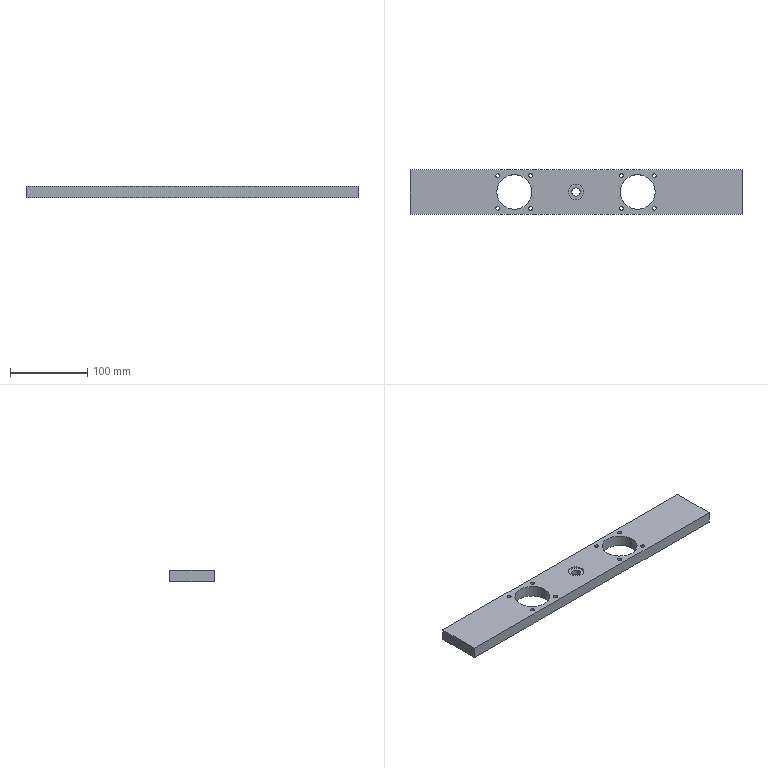Component | SolidWorks | Part19-1 | 1 solid | 31 faces | box 430 x 58 x 15 mm | volume 322167 mm3 | cylinder 24 | plane 7 | commonest cylinder face diameters 5 x16 45 x4 20 x2 11 x2
build123d program:
from build123d import *

# Parameters (mm, degrees)
SKETCH1_W                  = 430
SKETCH1_H                  = 58
BOSS_EXTRUDE1_DEPTH        = 15
SKETCH2_R                  = 5.5
CUT_EXTRUDE1_DEPTH         = 218.465
SKETCH3_R                  = 22.5
CUT_EXTRUDE2_DEPTH         = 218.465
M6_TAPPED_HOLE1_AT_2_COUNT = 2
M6_TAPPED_HOLE1_AT_2_PITCH = 42.426
M6_TAPPED_HOLE1_AT_3_COUNT = 2
M6_TAPPED_HOLE1_AT_3_PITCH = 42.426
M6_TAPPED_HOLE1_AT_4_COUNT = 2
M6_TAPPED_HOLE1_AT_4_PITCH = 60
SKETCH6_R                  = 10
CUT_EXTRUDE3_DEPTH         = 2


with BuildPart() as part:
    # Sketch1 → Boss-Extrude1 (new body)
    with BuildSketch(Plane.XY):
        Rectangle(SKETCH1_W, SKETCH1_H)
    extrude(amount=BOSS_EXTRUDE1_DEPTH)

    # Sketch2 → Cut-Extrude1 (cut, through all)
    with BuildSketch(Plane.XY.offset(15)):
        Circle(SKETCH2_R)
    extrude(amount=-CUT_EXTRUDE1_DEPTH, mode=Mode.SUBTRACT)

    # Sketch3 → Cut-Extrude2 (cut, through all)
    with BuildSketch(Plane.XY.offset(15)):
        with Locations((-80, 0)):
            Circle(SKETCH3_R)
    cut_extrude2 = extrude(amount=-CUT_EXTRUDE2_DEPTH, mode=Mode.SUBTRACT)

    # Sketch5 → M6 Tapped Hole1 (revolve, cut)
    with BuildSketch(Plane(origin=(-101.213, -21.213, 15), x_dir=(0, -1, 0), z_dir=(1, 0, 0))):
        Polygon((0, 0), (0, 16.502), (2.5, 15), (2.5, 0), align=None)
    m6_tapped_hole1 = revolve(axis=Axis((-101.213, -21.213, 21.35), (0, 0, -1)), mode=Mode.SUBTRACT)

    # M6 Tapped Hole1 at 2: M6 Tapped Hole1 ×2
    with Locations(*[(i * M6_TAPPED_HOLE1_AT_2_PITCH, 0, 0) for i in range(1, M6_TAPPED_HOLE1_AT_2_COUNT)]):
        add(m6_tapped_hole1, mode=Mode.SUBTRACT)

    # M6 Tapped Hole1 at 3: M6 Tapped Hole1 ×2
    with Locations(*[(0, i * M6_TAPPED_HOLE1_AT_3_PITCH, 0) for i in range(1, M6_TAPPED_HOLE1_AT_3_COUNT)]):
        add(m6_tapped_hole1, mode=Mode.SUBTRACT)

    # M6 Tapped Hole1 at 4: M6 Tapped Hole1 ×2
    with Locations(*[Vector(0.7071, 0.7071, 0) * (i * M6_TAPPED_HOLE1_AT_4_PITCH) for i in range(1, M6_TAPPED_HOLE1_AT_4_COUNT)]):
        add(m6_tapped_hole1, mode=Mode.SUBTRACT)

    # Mirror1: Cut-Extrude2, M6 Tapped Hole1 across plane
    add(cut_extrude2.mirror(Plane(origin=(0, 0, 0), x_dir=(0, 0, 1), z_dir=(1, 0, 0))), mode=Mode.SUBTRACT)
    add(m6_tapped_hole1.mirror(Plane(origin=(0, 0, 0), x_dir=(0, 0, 1), z_dir=(1, 0, 0))), mode=Mode.SUBTRACT)

    # Mirror1 copy 1 sketch → Mirror1 copy 1 (revolve, cut)
    with BuildSketch(Plane(origin=(58.787, -21.213, 15), x_dir=(0, -1, 0), z_dir=(-1, 0, 0))):
        Polygon((0, 0), (0, -16.502), (2.5, -15), (2.5, 0), align=None)
    revolve(axis=Axis((58.787, -21.213, 21.35), (0, 0, 1)), mode=Mode.SUBTRACT)

    # Mirror1 copy 2 sketch → Mirror1 copy 2 (revolve, cut)
    with BuildSketch(Plane(origin=(101.213, 21.213, 15), x_dir=(0, -1, 0), z_dir=(-1, 0, 0))):
        Polygon((0, 0), (0, -16.502), (2.5, -15), (2.5, 0), align=None)
    revolve(axis=Axis((101.213, 21.213, 21.35), (0, 0, 1)), mode=Mode.SUBTRACT)

    # Mirror1 copy 3 sketch → Mirror1 copy 3 (revolve, cut)
    with BuildSketch(Plane(origin=(58.787, 21.213, 15), x_dir=(0, -1, 0), z_dir=(-1, 0, 0))):
        Polygon((0, 0), (0, -16.502), (2.5, -15), (2.5, 0), align=None)
    revolve(axis=Axis((58.787, 21.213, 21.35), (0, 0, 1)), mode=Mode.SUBTRACT)

    # Sketch6 → Cut-Extrude3 (cut)
    with BuildSketch(Plane.XY.offset(15)):
        Circle(SKETCH6_R)
    extrude(amount=-CUT_EXTRUDE3_DEPTH, mode=Mode.SUBTRACT)


solid = part.part

# Placed as in the assembly
solid = solid.moved(Location((-87.007, -512, -285), (0, 0, 0)))
STEP:
#1=COLOUR_RGB('',0.7922,0.8196,0.9333);
#2=FILL_AREA_STYLE_COLOUR('',#1);
#3=FILL_AREA_STYLE('',(#2));
#4=SURFACE_STYLE_FILL_AREA(#3);
#5=SURFACE_SIDE_STYLE('',(#4));
#6=SURFACE_STYLE_USAGE(.BOTH.,#5);
#7=PRESENTATION_STYLE_ASSIGNMENT((#6));
#8=CARTESIAN_POINT('',(-3.819,-20.157,-10.709));
#9=VERTEX_POINT('',#8);
#10=CARTESIAN_POINT('',(-3.032,-20.157,-10.709));
#11=VERTEX_POINT('',#10);
#12=CARTESIAN_POINT('',(-3.425,-20.157,-10.709));
#13=DIRECTION('',(0.,0.,1.));
#14=DIRECTION('',(1.,0.,0.));
#15=AXIS2_PLACEMENT_3D('',#12,#13,#14);
#16=CIRCLE('',#15,0.3937);
#17=EDGE_CURVE('',#9,#11,#16,.T.);
#18=ORIENTED_EDGE('',*,*,#17,.F.);
#19=CARTESIAN_POINT('',(-3.819,-20.157,-10.63));
#20=VERTEX_POINT('',#19);
#21=CARTESIAN_POINT('',(-3.819,-20.157,-10.709));
#22=DIRECTION('',(0.,0.,1.));
#23=VECTOR('',#22,39.37);
#24=LINE('',#21,#23);
#25=EDGE_CURVE('',#9,#20,#24,.T.);
#26=ORIENTED_EDGE('',*,*,#25,.T.);
#27=CARTESIAN_POINT('',(-3.032,-20.157,-10.63));
#28=VERTEX_POINT('',#27);
#29=CARTESIAN_POINT('',(-3.425,-20.157,-10.63));
#30=DIRECTION('',(0.,0.,1.));
#31=DIRECTION('',(1.,0.,0.));
#32=AXIS2_PLACEMENT_3D('',#29,#30,#31);
#33=CIRCLE('',#32,0.3937);
#34=EDGE_CURVE('',#20,#28,#33,.T.);
#35=ORIENTED_EDGE('',*,*,#34,.T.);
#36=CARTESIAN_POINT('',(-3.032,-20.157,-10.709));
#37=DIRECTION('',(0.,0.,1.));
#38=VECTOR('',#37,39.37);
#39=LINE('',#36,#38);
#40=EDGE_CURVE('',#11,#28,#39,.T.);
#41=ORIENTED_EDGE('',*,*,#40,.F.);
#42=EDGE_LOOP('',(#18,#26,#35,#41));
#43=FACE_OUTER_BOUND('',#42,.T.);
#44=CARTESIAN_POINT('',(-3.425,-20.157,-10.709));
#45=DIRECTION('',(0.,0.,1.));
#46=DIRECTION('',(1.,0.,0.));
#47=AXIS2_PLACEMENT_3D('',#44,#45,#46);
#48=CYLINDRICAL_SURFACE('',#47,0.3937);
#49=ADVANCED_FACE('',(#43),#48,.F.);
#50=CARTESIAN_POINT('',(0.4609,-20.993,-11.22));
#51=VERTEX_POINT('',#50);
#52=CARTESIAN_POINT('',(0.6577,-20.993,-11.22));
#53=VERTEX_POINT('',#52);
#54=CARTESIAN_POINT('',(0.5593,-20.993,-11.22));
#55=DIRECTION('',(0.,0.,1.));
#56=DIRECTION('',(1.,0.,0.));
#57=AXIS2_PLACEMENT_3D('',#54,#55,#56);
#58=CIRCLE('',#57,0.09843);
#59=EDGE_CURVE('',#51,#53,#58,.T.);
#60=ORIENTED_EDGE('',*,*,#59,.F.);
#61=CARTESIAN_POINT('',(0.4609,-20.993,-10.63));
#62=VERTEX_POINT('',#61);
#63=CARTESIAN_POINT('',(0.4609,-20.993,-10.63));
#64=DIRECTION('',(0.,0.,1.));
#65=VECTOR('',#64,39.37);
#66=LINE('',#63,#65);
#67=EDGE_CURVE('',#51,#62,#66,.T.);
#68=ORIENTED_EDGE('',*,*,#67,.T.);
#69=CARTESIAN_POINT('',(0.6577,-20.993,-10.63));
#70=VERTEX_POINT('',#69);
#71=CARTESIAN_POINT('',(0.5593,-20.993,-10.63));
#72=DIRECTION('',(0.,0.,1.));
#73=DIRECTION('',(1.,0.,0.));
#74=AXIS2_PLACEMENT_3D('',#71,#72,#73);
#75=CIRCLE('',#74,0.09843);
#76=EDGE_CURVE('',#62,#70,#75,.T.);
#77=ORIENTED_EDGE('',*,*,#76,.T.);
#78=CARTESIAN_POINT('',(0.6577,-20.993,-10.63));
#79=DIRECTION('',(0.,0.,1.));
#80=VECTOR('',#79,39.37);
#81=LINE('',#78,#80);
#82=EDGE_CURVE('',#53,#70,#81,.T.);
#83=ORIENTED_EDGE('',*,*,#82,.F.);
#84=EDGE_LOOP('',(#60,#68,#77,#83));
#85=FACE_OUTER_BOUND('',#84,.T.);
#86=CARTESIAN_POINT('',(0.5593,-20.993,-10.63));
#87=DIRECTION('',(0.,0.,1.));
#88=DIRECTION('',(1.,0.,0.));
#89=AXIS2_PLACEMENT_3D('',#86,#87,#88);
#90=CYLINDRICAL_SURFACE('',#89,0.09843);
#91=ADVANCED_FACE('',(#85),#90,.F.);
#92=CARTESIAN_POINT('',(-1.209,-20.993,-11.22));
#93=VERTEX_POINT('',#92);
#94=CARTESIAN_POINT('',(-1.013,-20.993,-11.22));
#95=VERTEX_POINT('',#94);
#96=CARTESIAN_POINT('',(-1.111,-20.993,-11.22));
#97=DIRECTION('',(0.,0.,1.));
#98=DIRECTION('',(1.,0.,0.));
#99=AXIS2_PLACEMENT_3D('',#96,#97,#98);
#100=CIRCLE('',#99,0.09843);
#101=EDGE_CURVE('',#93,#95,#100,.T.);
#102=ORIENTED_EDGE('',*,*,#101,.F.);
#103=CARTESIAN_POINT('',(-1.209,-20.993,-10.63));
#104=VERTEX_POINT('',#103);
#105=CARTESIAN_POINT('',(-1.209,-20.993,-10.63));
#106=DIRECTION('',(0.,0.,1.));
#107=VECTOR('',#106,39.37);
#108=LINE('',#105,#107);
#109=EDGE_CURVE('',#93,#104,#108,.T.);
#110=ORIENTED_EDGE('',*,*,#109,.T.);
#111=CARTESIAN_POINT('',(-1.013,-20.993,-10.63));
#112=VERTEX_POINT('',#111);
#113=CARTESIAN_POINT('',(-1.111,-20.993,-10.63));
#114=DIRECTION('',(0.,0.,1.));
#115=DIRECTION('',(1.,0.,0.));
#116=AXIS2_PLACEMENT_3D('',#113,#114,#115);
#117=CIRCLE('',#116,0.09843);
#118=EDGE_CURVE('',#104,#112,#117,.T.);
#119=ORIENTED_EDGE('',*,*,#118,.T.);
#120=CARTESIAN_POINT('',(-1.013,-20.993,-10.63));
#121=DIRECTION('',(0.,0.,1.));
#122=VECTOR('',#121,39.37);
#123=LINE('',#120,#122);
#124=EDGE_CURVE('',#95,#112,#123,.T.);
#125=ORIENTED_EDGE('',*,*,#124,.F.);
#126=EDGE_LOOP('',(#102,#110,#119,#125));
#127=FACE_OUTER_BOUND('',#126,.T.);
#128=CARTESIAN_POINT('',(-1.111,-20.993,-10.63));
#129=DIRECTION('',(0.,0.,1.));
#130=DIRECTION('',(1.,0.,0.));
#131=AXIS2_PLACEMENT_3D('',#128,#129,#130);
#132=CYLINDRICAL_SURFACE('',#131,0.09843);
#133=ADVANCED_FACE('',(#127),#132,.F.);
#134=CARTESIAN_POINT('',(0.4609,-19.322,-11.22));
#135=VERTEX_POINT('',#134);
#136=CARTESIAN_POINT('',(0.6577,-19.322,-11.22));
#137=VERTEX_POINT('',#136);
#138=CARTESIAN_POINT('',(0.5593,-19.322,-11.22));
#139=DIRECTION('',(0.,0.,1.));
#140=DIRECTION('',(1.,0.,0.));
#141=AXIS2_PLACEMENT_3D('',#138,#139,#140);
#142=CIRCLE('',#141,0.09843);
#143=EDGE_CURVE('',#135,#137,#142,.T.);
#144=ORIENTED_EDGE('',*,*,#143,.F.);
#145=CARTESIAN_POINT('',(0.4609,-19.322,-10.63));
#146=VERTEX_POINT('',#145);
#147=CARTESIAN_POINT('',(0.4609,-19.322,-10.63));
#148=DIRECTION('',(0.,0.,1.));
#149=VECTOR('',#148,39.37);
#150=LINE('',#147,#149);
#151=EDGE_CURVE('',#135,#146,#150,.T.);
#152=ORIENTED_EDGE('',*,*,#151,.T.);
#153=CARTESIAN_POINT('',(0.6577,-19.322,-10.63));
#154=VERTEX_POINT('',#153);
#155=CARTESIAN_POINT('',(0.5593,-19.322,-10.63));
#156=DIRECTION('',(0.,0.,1.));
#157=DIRECTION('',(1.,0.,0.));
#158=AXIS2_PLACEMENT_3D('',#155,#156,#157);
#159=CIRCLE('',#158,0.09843);
#160=EDGE_CURVE('',#146,#154,#159,.T.);
#161=ORIENTED_EDGE('',*,*,#160,.T.);
#162=CARTESIAN_POINT('',(0.6577,-19.322,-10.63));
#163=DIRECTION('',(0.,0.,1.));
#164=VECTOR('',#163,39.37);
#165=LINE('',#162,#164);
#166=EDGE_CURVE('',#137,#154,#165,.T.);
#167=ORIENTED_EDGE('',*,*,#166,.F.);
#168=EDGE_LOOP('',(#144,#152,#161,#167));
#169=FACE_OUTER_BOUND('',#168,.T.);
#170=CARTESIAN_POINT('',(0.5593,-19.322,-10.63));
#171=DIRECTION('',(0.,0.,1.));
#172=DIRECTION('',(1.,0.,0.));
#173=AXIS2_PLACEMENT_3D('',#170,#171,#172);
#174=CYLINDRICAL_SURFACE('',#173,0.09843);
#175=ADVANCED_FACE('',(#169),#174,.F.);
#176=CARTESIAN_POINT('',(-1.209,-19.322,-11.22));
#177=VERTEX_POINT('',#176);
#178=CARTESIAN_POINT('',(-1.013,-19.322,-11.22));
#179=VERTEX_POINT('',#178);
#180=CARTESIAN_POINT('',(-1.111,-19.322,-11.22));
#181=DIRECTION('',(0.,0.,1.));
#182=DIRECTION('',(1.,0.,0.));
#183=AXIS2_PLACEMENT_3D('',#180,#181,#182);
#184=CIRCLE('',#183,0.09843);
#185=EDGE_CURVE('',#177,#179,#184,.T.);
#186=ORIENTED_EDGE('',*,*,#185,.F.);
#187=CARTESIAN_POINT('',(-1.209,-19.322,-10.63));
#188=VERTEX_POINT('',#187);
#189=CARTESIAN_POINT('',(-1.209,-19.322,-10.63));
#190=DIRECTION('',(0.,0.,1.));
#191=VECTOR('',#190,39.37);
#192=LINE('',#189,#191);
#193=EDGE_CURVE('',#177,#188,#192,.T.);
#194=ORIENTED_EDGE('',*,*,#193,.T.);
#195=CARTESIAN_POINT('',(-1.013,-19.322,-10.63));
#196=VERTEX_POINT('',#195);
#197=CARTESIAN_POINT('',(-1.111,-19.322,-10.63));
#198=DIRECTION('',(0.,0.,1.));
#199=DIRECTION('',(1.,0.,0.));
#200=AXIS2_PLACEMENT_3D('',#197,#198,#199);
#201=CIRCLE('',#200,0.09843);
#202=EDGE_CURVE('',#188,#196,#201,.T.);
#203=ORIENTED_EDGE('',*,*,#202,.T.);
#204=CARTESIAN_POINT('',(-1.013,-19.322,-10.63));
#205=DIRECTION('',(0.,0.,1.));
#206=VECTOR('',#205,39.37);
#207=LINE('',#204,#206);
#208=EDGE_CURVE('',#179,#196,#207,.T.);
#209=ORIENTED_EDGE('',*,*,#208,.F.);
#210=EDGE_LOOP('',(#186,#194,#203,#209));
#211=FACE_OUTER_BOUND('',#210,.T.);
#212=CARTESIAN_POINT('',(-1.111,-19.322,-10.63));
#213=DIRECTION('',(0.,0.,1.));
#214=DIRECTION('',(1.,0.,0.));
#215=AXIS2_PLACEMENT_3D('',#212,#213,#214);
#216=CYLINDRICAL_SURFACE('',#215,0.09843);
#217=ADVANCED_FACE('',(#211),#216,.F.);
#218=CARTESIAN_POINT('',(0.61,-20.157,-11.22));
#219=VERTEX_POINT('',#218);
#220=CARTESIAN_POINT('',(-1.162,-20.157,-11.22));
#221=VERTEX_POINT('',#220);
#222=CARTESIAN_POINT('',(-0.2759,-20.157,-11.22));
#223=DIRECTION('',(0.,0.,-1.));
#224=DIRECTION('',(-1.,0.,0.));
#225=AXIS2_PLACEMENT_3D('',#222,#223,#224);
#226=CIRCLE('',#225,0.8858);
#227=EDGE_CURVE('',#219,#221,#226,.T.);
#228=ORIENTED_EDGE('',*,*,#227,.T.);
#229=CARTESIAN_POINT('',(-1.162,-20.157,-10.63));
#230=VERTEX_POINT('',#229);
#231=CARTESIAN_POINT('',(-1.162,-20.157,-11.22));
#232=DIRECTION('',(0.,0.,1.));
#233=VECTOR('',#232,39.37);
#234=LINE('',#231,#233);
#235=EDGE_CURVE('',#221,#230,#234,.T.);
#236=ORIENTED_EDGE('',*,*,#235,.T.);
#237=CARTESIAN_POINT('',(0.61,-20.157,-10.63));
#238=VERTEX_POINT('',#237);
#239=CARTESIAN_POINT('',(-0.2759,-20.157,-10.63));
#240=DIRECTION('',(0.,0.,-1.));
#241=DIRECTION('',(-1.,0.,0.));
#242=AXIS2_PLACEMENT_3D('',#239,#240,#241);
#243=CIRCLE('',#242,0.8858);
#244=EDGE_CURVE('',#238,#230,#243,.T.);
#245=ORIENTED_EDGE('',*,*,#244,.F.);
#246=CARTESIAN_POINT('',(0.61,-20.157,-11.22));
#247=DIRECTION('',(0.,0.,1.));
#248=VECTOR('',#247,39.37);
#249=LINE('',#246,#248);
#250=EDGE_CURVE('',#219,#238,#249,.T.);
#251=ORIENTED_EDGE('',*,*,#250,.F.);
#252=EDGE_LOOP('',(#228,#236,#245,#251));
#253=FACE_OUTER_BOUND('',#252,.T.);
#254=CARTESIAN_POINT('',(-0.2759,-20.157,-11.22));
#255=DIRECTION('',(0.,0.,1.));
#256=DIRECTION('',(1.,0.,0.));
#257=AXIS2_PLACEMENT_3D('',#254,#255,#256);
#258=CYLINDRICAL_SURFACE('',#257,0.8858);
#259=ADVANCED_FACE('',(#253),#258,.F.);
#260=CARTESIAN_POINT('',(-7.509,-20.993,-11.22));
#261=VERTEX_POINT('',#260);
#262=CARTESIAN_POINT('',(-7.312,-20.993,-11.22));
#263=VERTEX_POINT('',#262);
#264=CARTESIAN_POINT('',(-7.41,-20.993,-11.22));
#265=DIRECTION('',(0.,0.,1.));
#266=DIRECTION('',(1.,0.,0.));
#267=AXIS2_PLACEMENT_3D('',#264,#265,#266);
#268=CIRCLE('',#267,0.09843);
#269=EDGE_CURVE('',#261,#263,#268,.T.);
#270=ORIENTED_EDGE('',*,*,#269,.F.);
#271=CARTESIAN_POINT('',(-7.509,-20.993,-10.63));
#272=VERTEX_POINT('',#271);
#273=CARTESIAN_POINT('',(-7.509,-20.993,-10.63));
#274=DIRECTION('',(0.,0.,1.));
#275=VECTOR('',#274,39.37);
#276=LINE('',#273,#275);
#277=EDGE_CURVE('',#261,#272,#276,.T.);
#278=ORIENTED_EDGE('',*,*,#277,.T.);
#279=CARTESIAN_POINT('',(-7.312,-20.993,-10.63));
#280=VERTEX_POINT('',#279);
#281=CARTESIAN_POINT('',(-7.41,-20.993,-10.63));
#282=DIRECTION('',(0.,0.,1.));
#283=DIRECTION('',(1.,0.,0.));
#284=AXIS2_PLACEMENT_3D('',#281,#282,#283);
#285=CIRCLE('',#284,0.09843);
#286=EDGE_CURVE('',#272,#280,#285,.T.);
#287=ORIENTED_EDGE('',*,*,#286,.T.);
#288=CARTESIAN_POINT('',(-7.312,-20.993,-10.63));
#289=DIRECTION('',(0.,0.,1.));
#290=VECTOR('',#289,39.37);
#291=LINE('',#288,#290);
#292=EDGE_CURVE('',#263,#280,#291,.T.);
#293=ORIENTED_EDGE('',*,*,#292,.F.);
#294=EDGE_LOOP('',(#270,#278,#287,#293));
#295=FACE_OUTER_BOUND('',#294,.T.);
#296=CARTESIAN_POINT('',(-7.41,-20.993,-10.63));
#297=DIRECTION('',(0.,0.,1.));
#298=DIRECTION('',(1.,0.,0.));
#299=AXIS2_PLACEMENT_3D('',#296,#297,#298);
#300=CYLINDRICAL_SURFACE('',#299,0.09843);
#301=ADVANCED_FACE('',(#295),#300,.F.);
#302=CARTESIAN_POINT('',(-5.838,-20.993,-11.22));
#303=VERTEX_POINT('',#302);
#304=CARTESIAN_POINT('',(-5.641,-20.993,-11.22));
#305=VERTEX_POINT('',#304);
#306=CARTESIAN_POINT('',(-5.74,-20.993,-11.22));
#307=DIRECTION('',(0.,0.,1.));
#308=DIRECTION('',(1.,0.,0.));
#309=AXIS2_PLACEMENT_3D('',#306,#307,#308);
#310=CIRCLE('',#309,0.09843);
#311=EDGE_CURVE('',#303,#305,#310,.T.);
#312=ORIENTED_EDGE('',*,*,#311,.F.);
#313=CARTESIAN_POINT('',(-5.838,-20.993,-10.63));
#314=VERTEX_POINT('',#313);
#315=CARTESIAN_POINT('',(-5.838,-20.993,-10.63));
#316=DIRECTION('',(0.,0.,1.));
#317=VECTOR('',#316,39.37);
#318=LINE('',#315,#317);
#319=EDGE_CURVE('',#303,#314,#318,.T.);
#320=ORIENTED_EDGE('',*,*,#319,.T.);
#321=CARTESIAN_POINT('',(-5.641,-20.993,-10.63));
#322=VERTEX_POINT('',#321);
#323=CARTESIAN_POINT('',(-5.74,-20.993,-10.63));
#324=DIRECTION('',(0.,0.,1.));
#325=DIRECTION('',(1.,0.,0.));
#326=AXIS2_PLACEMENT_3D('',#323,#324,#325);
#327=CIRCLE('',#326,0.09843);
#328=EDGE_CURVE('',#314,#322,#327,.T.);
#329=ORIENTED_EDGE('',*,*,#328,.T.);
#330=CARTESIAN_POINT('',(-5.641,-20.993,-10.63));
#331=DIRECTION('',(0.,0.,1.));
#332=VECTOR('',#331,39.37);
#333=LINE('',#330,#332);
#334=EDGE_CURVE('',#305,#322,#333,.T.);
#335=ORIENTED_EDGE('',*,*,#334,.F.);
#336=EDGE_LOOP('',(#312,#320,#329,#335));
#337=FACE_OUTER_BOUND('',#336,.T.);
#338=CARTESIAN_POINT('',(-5.74,-20.993,-10.63));
#339=DIRECTION('',(0.,0.,1.));
#340=DIRECTION('',(1.,0.,0.));
#341=AXIS2_PLACEMENT_3D('',#338,#339,#340);
#342=CYLINDRICAL_SURFACE('',#341,0.09843);
#343=ADVANCED_FACE('',(#337),#342,.F.);
#344=CARTESIAN_POINT('',(-7.509,-19.322,-11.22));
#345=VERTEX_POINT('',#344);
#346=CARTESIAN_POINT('',(-7.312,-19.322,-11.22));
#347=VERTEX_POINT('',#346);
#348=CARTESIAN_POINT('',(-7.41,-19.322,-11.22));
#349=DIRECTION('',(0.,0.,1.));
#350=DIRECTION('',(1.,0.,0.));
#351=AXIS2_PLACEMENT_3D('',#348,#349,#350);
#352=CIRCLE('',#351,0.09843);
#353=EDGE_CURVE('',#345,#347,#352,.T.);
#354=ORIENTED_EDGE('',*,*,#353,.F.);
#355=CARTESIAN_POINT('',(-7.509,-19.322,-10.63));
#356=VERTEX_POINT('',#355);
#357=CARTESIAN_POINT('',(-7.509,-19.322,-10.63));
#358=DIRECTION('',(0.,0.,1.));
#359=VECTOR('',#358,39.37);
#360=LINE('',#357,#359);
#361=EDGE_CURVE('',#345,#356,#360,.T.);
#362=ORIENTED_EDGE('',*,*,#361,.T.);
#363=CARTESIAN_POINT('',(-7.312,-19.322,-10.63));
#364=VERTEX_POINT('',#363);
#365=CARTESIAN_POINT('',(-7.41,-19.322,-10.63));
#366=DIRECTION('',(0.,0.,1.));
#367=DIRECTION('',(1.,0.,0.));
#368=AXIS2_PLACEMENT_3D('',#365,#366,#367);
#369=CIRCLE('',#368,0.09843);
#370=EDGE_CURVE('',#356,#364,#369,.T.);
#371=ORIENTED_EDGE('',*,*,#370,.T.);
#372=CARTESIAN_POINT('',(-7.312,-19.322,-10.63));
#373=DIRECTION('',(0.,0.,1.));
#374=VECTOR('',#373,39.37);
#375=LINE('',#372,#374);
#376=EDGE_CURVE('',#347,#364,#375,.T.);
#377=ORIENTED_EDGE('',*,*,#376,.F.);
#378=EDGE_LOOP('',(#354,#362,#371,#377));
#379=FACE_OUTER_BOUND('',#378,.T.);
#380=CARTESIAN_POINT('',(-7.41,-19.322,-10.63));
#381=DIRECTION('',(0.,0.,1.));
#382=DIRECTION('',(1.,0.,0.));
#383=AXIS2_PLACEMENT_3D('',#380,#381,#382);
#384=CYLINDRICAL_SURFACE('',#383,0.09843);
#385=ADVANCED_FACE('',(#379),#384,.F.);
#386=CARTESIAN_POINT('',(-5.838,-19.322,-11.22));
#387=VERTEX_POINT('',#386);
#388=CARTESIAN_POINT('',(-5.641,-19.322,-11.22));
#389=VERTEX_POINT('',#388);
#390=CARTESIAN_POINT('',(-5.74,-19.322,-11.22));
#391=DIRECTION('',(0.,0.,1.));
#392=DIRECTION('',(1.,0.,0.));
#393=AXIS2_PLACEMENT_3D('',#390,#391,#392);
#394=CIRCLE('',#393,0.09843);
#395=EDGE_CURVE('',#387,#389,#394,.T.);
#396=ORIENTED_EDGE('',*,*,#395,.F.);
#397=CARTESIAN_POINT('',(-5.838,-19.322,-10.63));
#398=VERTEX_POINT('',#397);
#399=CARTESIAN_POINT('',(-5.838,-19.322,-10.63));
#400=DIRECTION('',(0.,0.,1.));
#401=VECTOR('',#400,39.37);
#402=LINE('',#399,#401);
#403=EDGE_CURVE('',#387,#398,#402,.T.);
#404=ORIENTED_EDGE('',*,*,#403,.T.);
#405=CARTESIAN_POINT('',(-5.641,-19.322,-10.63));
#406=VERTEX_POINT('',#405);
#407=CARTESIAN_POINT('',(-5.74,-19.322,-10.63));
#408=DIRECTION('',(0.,0.,1.));
#409=DIRECTION('',(1.,0.,0.));
#410=AXIS2_PLACEMENT_3D('',#407,#408,#409);
#411=CIRCLE('',#410,0.09843);
#412=EDGE_CURVE('',#398,#406,#411,.T.);
#413=ORIENTED_EDGE('',*,*,#412,.T.);
#414=CARTESIAN_POINT('',(-5.641,-19.322,-10.63));
#415=DIRECTION('',(0.,0.,1.));
#416=VECTOR('',#415,39.37);
#417=LINE('',#414,#416);
#418=EDGE_CURVE('',#389,#406,#417,.T.);
#419=ORIENTED_EDGE('',*,*,#418,.F.);
#420=EDGE_LOOP('',(#396,#404,#413,#419));
#421=FACE_OUTER_BOUND('',#420,.T.);
#422=CARTESIAN_POINT('',(-5.74,-19.322,-10.63));
#423=DIRECTION('',(0.,0.,1.));
#424=DIRECTION('',(1.,0.,0.));
#425=AXIS2_PLACEMENT_3D('',#422,#423,#424);
#426=CYLINDRICAL_SURFACE('',#425,0.09843);
#427=ADVANCED_FACE('',(#421),#426,.F.);
#428=CARTESIAN_POINT('',(-7.461,-20.157,-11.22));
#429=VERTEX_POINT('',#428);
#430=CARTESIAN_POINT('',(-5.689,-20.157,-11.22));
#431=VERTEX_POINT('',#430);
#432=CARTESIAN_POINT('',(-6.575,-20.157,-11.22));
#433=DIRECTION('',(0.,0.,1.));
#434=DIRECTION('',(1.,0.,0.));
#435=AXIS2_PLACEMENT_3D('',#432,#433,#434);
#436=CIRCLE('',#435,0.8858);
#437=EDGE_CURVE('',#429,#431,#436,.T.);
#438=ORIENTED_EDGE('',*,*,#437,.F.);
#439=CARTESIAN_POINT('',(-7.461,-20.157,-10.63));
#440=VERTEX_POINT('',#439);
#441=CARTESIAN_POINT('',(-7.461,-20.157,-11.22));
#442=DIRECTION('',(0.,0.,1.));
#443=VECTOR('',#442,39.37);
#444=LINE('',#441,#443);
#445=EDGE_CURVE('',#429,#440,#444,.T.);
#446=ORIENTED_EDGE('',*,*,#445,.T.);
#447=CARTESIAN_POINT('',(-5.689,-20.157,-10.63));
#448=VERTEX_POINT('',#447);
#449=CARTESIAN_POINT('',(-6.575,-20.157,-10.63));
#450=DIRECTION('',(0.,0.,1.));
#451=DIRECTION('',(1.,0.,0.));
#452=AXIS2_PLACEMENT_3D('',#449,#450,#451);
#453=CIRCLE('',#452,0.8858);
#454=EDGE_CURVE('',#440,#448,#453,.T.);
#455=ORIENTED_EDGE('',*,*,#454,.T.);
#456=CARTESIAN_POINT('',(-5.689,-20.157,-11.22));
#457=DIRECTION('',(0.,0.,1.));
#458=VECTOR('',#457,39.37);
#459=LINE('',#456,#458);
#460=EDGE_CURVE('',#431,#448,#459,.T.);
#461=ORIENTED_EDGE('',*,*,#460,.F.);
#462=EDGE_LOOP('',(#438,#446,#455,#461));
#463=FACE_OUTER_BOUND('',#462,.T.);
#464=CARTESIAN_POINT('',(-6.575,-20.157,-11.22));
#465=DIRECTION('',(0.,0.,1.));
#466=DIRECTION('',(1.,0.,0.));
#467=AXIS2_PLACEMENT_3D('',#464,#465,#466);
#468=CYLINDRICAL_SURFACE('',#467,0.8858);
#469=ADVANCED_FACE('',(#463),#468,.F.);
#470=CARTESIAN_POINT('',(-3.642,-20.157,-11.22));
#471=VERTEX_POINT('',#470);
#472=CARTESIAN_POINT('',(-3.209,-20.157,-11.22));
#473=VERTEX_POINT('',#472);
#474=CARTESIAN_POINT('',(-3.425,-20.157,-11.22));
#475=DIRECTION('',(0.,0.,1.));
#476=DIRECTION('',(1.,0.,0.));
#477=AXIS2_PLACEMENT_3D('',#474,#475,#476);
#478=CIRCLE('',#477,0.2165);
#479=EDGE_CURVE('',#471,#473,#478,.T.);
#480=ORIENTED_EDGE('',*,*,#479,.F.);
#481=CARTESIAN_POINT('',(-3.642,-20.157,-10.709));
#482=VERTEX_POINT('',#481);
#483=CARTESIAN_POINT('',(-3.642,-20.157,-11.22));
#484=DIRECTION('',(0.,0.,1.));
#485=VECTOR('',#484,39.37);
#486=LINE('',#483,#485);
#487=EDGE_CURVE('',#471,#482,#486,.T.);
#488=ORIENTED_EDGE('',*,*,#487,.T.);
#489=CARTESIAN_POINT('',(-3.209,-20.157,-10.709));
#490=VERTEX_POINT('',#489);
#491=CARTESIAN_POINT('',(-3.425,-20.157,-10.709));
#492=DIRECTION('',(0.,0.,-1.));
#493=DIRECTION('',(1.,0.,0.));
#494=AXIS2_PLACEMENT_3D('',#491,#492,#493);
#495=CIRCLE('',#494,0.2165);
#496=EDGE_CURVE('',#490,#482,#495,.T.);
#497=ORIENTED_EDGE('',*,*,#496,.F.);
#498=CARTESIAN_POINT('',(-3.209,-20.157,-11.22));
#499=DIRECTION('',(0.,0.,1.));
#500=VECTOR('',#499,39.37);
#501=LINE('',#498,#500);
#502=EDGE_CURVE('',#473,#490,#501,.T.);
#503=ORIENTED_EDGE('',*,*,#502,.F.);
#504=EDGE_LOOP('',(#480,#488,#497,#503));
#505=FACE_OUTER_BOUND('',#504,.T.);
#506=CARTESIAN_POINT('',(-3.425,-20.157,-11.22));
#507=DIRECTION('',(0.,0.,1.));
#508=DIRECTION('',(1.,0.,0.));
#509=AXIS2_PLACEMENT_3D('',#506,#507,#508);
#510=CYLINDRICAL_SURFACE('',#509,0.2165);
#511=ADVANCED_FACE('',(#505),#510,.F.);
#512=ORIENTED_EDGE('',*,*,#487,.F.);
#513=CARTESIAN_POINT('',(-3.425,-20.157,-11.22));
#514=DIRECTION('',(0.,0.,1.));
#515=DIRECTION('',(1.,0.,0.));
#516=AXIS2_PLACEMENT_3D('',#513,#514,#515);
#517=CIRCLE('',#516,0.2165);
#518=EDGE_CURVE('',#473,#471,#517,.T.);
#519=ORIENTED_EDGE('',*,*,#518,.F.);
#520=ORIENTED_EDGE('',*,*,#502,.T.);
#521=CARTESIAN_POINT('',(-3.425,-20.157,-10.709));
#522=DIRECTION('',(0.,0.,-1.));
#523=DIRECTION('',(1.,0.,0.));
#524=AXIS2_PLACEMENT_3D('',#521,#522,#523);
#525=CIRCLE('',#524,0.2165);
#526=EDGE_CURVE('',#482,#490,#525,.T.);
#527=ORIENTED_EDGE('',*,*,#526,.F.);
#528=EDGE_LOOP('',(#512,#519,#520,#527));
#529=FACE_OUTER_BOUND('',#528,.T.);
#530=CARTESIAN_POINT('',(-3.425,-20.157,-11.22));
#531=DIRECTION('',(0.,0.,1.));
#532=DIRECTION('',(1.,0.,0.));
#533=AXIS2_PLACEMENT_3D('',#530,#531,#532);
#534=CYLINDRICAL_SURFACE('',#533,0.2165);
#535=ADVANCED_FACE('',(#529),#534,.F.);
#536=CARTESIAN_POINT('',(5.039,-21.299,-11.22));
#537=VERTEX_POINT('',#536);
#538=CARTESIAN_POINT('',(5.039,-19.016,-11.22));
#539=VERTEX_POINT('',#538);
#540=CARTESIAN_POINT('',(5.039,-21.299,-11.22));
#541=DIRECTION('',(0.,1.,0.));
#542=VECTOR('',#541,39.37);
#543=LINE('',#540,#542);
#544=EDGE_CURVE('',#537,#539,#543,.T.);
#545=ORIENTED_EDGE('',*,*,#544,.T.);
#546=CARTESIAN_POINT('',(5.039,-19.016,-10.63));
#547=VERTEX_POINT('',#546);
#548=CARTESIAN_POINT('',(5.039,-19.016,-10.63));
#549=DIRECTION('',(0.,0.,-1.));
#550=VECTOR('',#549,39.37);
#551=LINE('',#548,#550);
#552=EDGE_CURVE('',#547,#539,#551,.T.);
#553=ORIENTED_EDGE('',*,*,#552,.F.);
#554=CARTESIAN_POINT('',(5.039,-21.299,-10.63));
#555=VERTEX_POINT('',#554);
#556=CARTESIAN_POINT('',(5.039,-21.299,-10.63));
#557=DIRECTION('',(0.,1.,0.));
#558=VECTOR('',#557,39.37);
#559=LINE('',#556,#558);
#560=EDGE_CURVE('',#555,#547,#559,.T.);
#561=ORIENTED_EDGE('',*,*,#560,.F.);
#562=CARTESIAN_POINT('',(5.039,-21.299,-10.63));
#563=DIRECTION('',(0.,0.,-1.));
#564=VECTOR('',#563,39.37);
#565=LINE('',#562,#564);
#566=EDGE_CURVE('',#555,#537,#565,.T.);
#567=ORIENTED_EDGE('',*,*,#566,.T.);
#568=EDGE_LOOP('',(#545,#553,#561,#567));
#569=FACE_OUTER_BOUND('',#568,.T.);
#570=CARTESIAN_POINT('',(5.039,-21.299,-10.63));
#571=DIRECTION('',(-1.,0.,0.));
#572=DIRECTION('',(0.,0.,1.));
#573=AXIS2_PLACEMENT_3D('',#570,#571,#572);
#574=PLANE('',#573);
#575=ADVANCED_FACE('',(#569),#574,.F.);
#576=CARTESIAN_POINT('',(-11.89,-19.016,-11.22));
#577=VERTEX_POINT('',#576);
#578=CARTESIAN_POINT('',(-11.89,-19.016,-11.22));
#579=DIRECTION('',(-1.,0.,0.));
#580=VECTOR('',#579,39.37);
#581=LINE('',#578,#580);
#582=EDGE_CURVE('',#539,#577,#581,.T.);
#583=ORIENTED_EDGE('',*,*,#582,.T.);
#584=CARTESIAN_POINT('',(-11.89,-19.016,-10.63));
#585=VERTEX_POINT('',#584);
#586=CARTESIAN_POINT('',(-11.89,-19.016,-10.63));
#587=DIRECTION('',(0.,0.,-1.));
#588=VECTOR('',#587,39.37);
#589=LINE('',#586,#588);
#590=EDGE_CURVE('',#585,#577,#589,.T.);
#591=ORIENTED_EDGE('',*,*,#590,.F.);
#592=CARTESIAN_POINT('',(-11.89,-19.016,-10.63));
#593=DIRECTION('',(-1.,0.,0.));
#594=VECTOR('',#593,39.37);
#595=LINE('',#592,#594);
#596=EDGE_CURVE('',#547,#585,#595,.T.);
#597=ORIENTED_EDGE('',*,*,#596,.F.);
#598=ORIENTED_EDGE('',*,*,#552,.T.);
#599=EDGE_LOOP('',(#583,#591,#597,#598));
#600=FACE_OUTER_BOUND('',#599,.T.);
#601=CARTESIAN_POINT('',(-11.89,-19.016,-10.63));
#602=DIRECTION('',(0.,-1.,0.));
#603=DIRECTION('',(0.,0.,-1.));
#604=AXIS2_PLACEMENT_3D('',#601,#602,#603);
#605=PLANE('',#604);
#606=ADVANCED_FACE('',(#600),#605,.F.);
#607=CARTESIAN_POINT('',(-11.89,-21.299,-11.22));
#608=VERTEX_POINT('',#607);
#609=CARTESIAN_POINT('',(-11.89,-21.299,-11.22));
#610=DIRECTION('',(0.,-1.,0.));
#611=VECTOR('',#610,39.37);
#612=LINE('',#609,#611);
#613=EDGE_CURVE('',#577,#608,#612,.T.);
#614=ORIENTED_EDGE('',*,*,#613,.T.);
#615=CARTESIAN_POINT('',(-11.89,-21.299,-10.63));
#616=VERTEX_POINT('',#615);
#617=CARTESIAN_POINT('',(-11.89,-21.299,-10.63));
#618=DIRECTION('',(0.,0.,-1.));
#619=VECTOR('',#618,39.37);
#620=LINE('',#617,#619);
#621=EDGE_CURVE('',#616,#608,#620,.T.);
#622=ORIENTED_EDGE('',*,*,#621,.F.);
#623=CARTESIAN_POINT('',(-11.89,-21.299,-10.63));
#624=DIRECTION('',(0.,-1.,0.));
#625=VECTOR('',#624,39.37);
#626=LINE('',#623,#625);
#627=EDGE_CURVE('',#585,#616,#626,.T.);
#628=ORIENTED_EDGE('',*,*,#627,.F.);
#629=ORIENTED_EDGE('',*,*,#590,.T.);
#630=EDGE_LOOP('',(#614,#622,#628,#629));
#631=FACE_OUTER_BOUND('',#630,.T.);
#632=CARTESIAN_POINT('',(-11.89,-21.299,-10.63));
#633=DIRECTION('',(1.,0.,0.));
#634=DIRECTION('',(0.,0.,-1.));
#635=AXIS2_PLACEMENT_3D('',#632,#633,#634);
#636=PLANE('',#635);
#637=ADVANCED_FACE('',(#631),#636,.F.);
#638=CARTESIAN_POINT('',(-11.89,-21.299,-11.22));
#639=DIRECTION('',(1.,0.,0.));
#640=VECTOR('',#639,39.37);
#641=LINE('',#638,#640);
#642=EDGE_CURVE('',#608,#537,#641,.T.);
#643=ORIENTED_EDGE('',*,*,#642,.T.);
#644=ORIENTED_EDGE('',*,*,#566,.F.);
#645=CARTESIAN_POINT('',(-11.89,-21.299,-10.63));
#646=DIRECTION('',(1.,0.,0.));
#647=VECTOR('',#646,39.37);
#648=LINE('',#645,#647);
#649=EDGE_CURVE('',#616,#555,#648,.T.);
#650=ORIENTED_EDGE('',*,*,#649,.F.);
#651=ORIENTED_EDGE('',*,*,#621,.T.);
#652=EDGE_LOOP('',(#643,#644,#650,#651));
#653=FACE_OUTER_BOUND('',#652,.T.);
#654=CARTESIAN_POINT('',(-11.89,-21.299,-10.63));
#655=DIRECTION('',(0.,1.,0.));
#656=DIRECTION('',(0.,0.,1.));
#657=AXIS2_PLACEMENT_3D('',#654,#655,#656);
#658=PLANE('',#657);
#659=ADVANCED_FACE('',(#653),#658,.F.);
#660=CARTESIAN_POINT('',(-3.425,-20.157,-10.63));
#661=DIRECTION('',(0.,0.,1.));
#662=DIRECTION('',(1.,0.,0.));
#663=AXIS2_PLACEMENT_3D('',#660,#661,#662);
#664=CIRCLE('',#663,0.3937);
#665=EDGE_CURVE('',#28,#20,#664,.T.);
#666=ORIENTED_EDGE('',*,*,#665,.F.);
#667=ORIENTED_EDGE('',*,*,#34,.F.);
#668=EDGE_LOOP('',(#666,#667));
#669=FACE_BOUND('',#668,.T.);
#670=CARTESIAN_POINT('',(0.5593,-20.993,-10.63));
#671=DIRECTION('',(0.,0.,1.));
#672=DIRECTION('',(1.,0.,0.));
#673=AXIS2_PLACEMENT_3D('',#670,#671,#672);
#674=CIRCLE('',#673,0.09843);
#675=EDGE_CURVE('',#70,#62,#674,.T.);
#676=ORIENTED_EDGE('',*,*,#675,.F.);
#677=ORIENTED_EDGE('',*,*,#76,.F.);
#678=EDGE_LOOP('',(#676,#677));
#679=FACE_BOUND('',#678,.T.);
#680=CARTESIAN_POINT('',(-1.111,-20.993,-10.63));
#681=DIRECTION('',(0.,0.,1.));
#682=DIRECTION('',(1.,0.,0.));
#683=AXIS2_PLACEMENT_3D('',#680,#681,#682);
#684=CIRCLE('',#683,0.09843);
#685=EDGE_CURVE('',#112,#104,#684,.T.);
#686=ORIENTED_EDGE('',*,*,#685,.F.);
#687=ORIENTED_EDGE('',*,*,#118,.F.);
#688=EDGE_LOOP('',(#686,#687));
#689=FACE_BOUND('',#688,.T.);
#690=CARTESIAN_POINT('',(0.5593,-19.322,-10.63));
#691=DIRECTION('',(0.,0.,1.));
#692=DIRECTION('',(1.,0.,0.));
#693=AXIS2_PLACEMENT_3D('',#690,#691,#692);
#694=CIRCLE('',#693,0.09843);
#695=EDGE_CURVE('',#154,#146,#694,.T.);
#696=ORIENTED_EDGE('',*,*,#695,.F.);
#697=ORIENTED_EDGE('',*,*,#160,.F.);
#698=EDGE_LOOP('',(#696,#697));
#699=FACE_BOUND('',#698,.T.);
#700=CARTESIAN_POINT('',(-1.111,-19.322,-10.63));
#701=DIRECTION('',(0.,0.,1.));
#702=DIRECTION('',(1.,0.,0.));
#703=AXIS2_PLACEMENT_3D('',#700,#701,#702);
#704=CIRCLE('',#703,0.09843);
#705=EDGE_CURVE('',#196,#188,#704,.T.);
#706=ORIENTED_EDGE('',*,*,#705,.F.);
#707=ORIENTED_EDGE('',*,*,#202,.F.);
#708=EDGE_LOOP('',(#706,#707));
#709=FACE_BOUND('',#708,.T.);
#710=ORIENTED_EDGE('',*,*,#244,.T.);
#711=CARTESIAN_POINT('',(-0.2759,-20.157,-10.63));
#712=DIRECTION('',(0.,0.,-1.));
#713=DIRECTION('',(-1.,0.,0.));
#714=AXIS2_PLACEMENT_3D('',#711,#712,#713);
#715=CIRCLE('',#714,0.8858);
#716=EDGE_CURVE('',#230,#238,#715,.T.);
#717=ORIENTED_EDGE('',*,*,#716,.T.);
#718=EDGE_LOOP('',(#710,#717));
#719=FACE_BOUND('',#718,.T.);
#720=CARTESIAN_POINT('',(-7.41,-20.993,-10.63));
#721=DIRECTION('',(0.,0.,1.));
#722=DIRECTION('',(1.,0.,0.));
#723=AXIS2_PLACEMENT_3D('',#720,#721,#722);
#724=CIRCLE('',#723,0.09843);
#725=EDGE_CURVE('',#280,#272,#724,.T.);
#726=ORIENTED_EDGE('',*,*,#725,.F.);
#727=ORIENTED_EDGE('',*,*,#286,.F.);
#728=EDGE_LOOP('',(#726,#727));
#729=FACE_BOUND('',#728,.T.);
#730=CARTESIAN_POINT('',(-5.74,-20.993,-10.63));
#731=DIRECTION('',(0.,0.,1.));
#732=DIRECTION('',(1.,0.,0.));
#733=AXIS2_PLACEMENT_3D('',#730,#731,#732);
#734=CIRCLE('',#733,0.09843);
#735=EDGE_CURVE('',#322,#314,#734,.T.);
#736=ORIENTED_EDGE('',*,*,#735,.F.);
#737=ORIENTED_EDGE('',*,*,#328,.F.);
#738=EDGE_LOOP('',(#736,#737));
#739=FACE_BOUND('',#738,.T.);
#740=CARTESIAN_POINT('',(-7.41,-19.322,-10.63));
#741=DIRECTION('',(0.,0.,1.));
#742=DIRECTION('',(1.,0.,0.));
#743=AXIS2_PLACEMENT_3D('',#740,#741,#742);
#744=CIRCLE('',#743,0.09843);
#745=EDGE_CURVE('',#364,#356,#744,.T.);
#746=ORIENTED_EDGE('',*,*,#745,.F.);
#747=ORIENTED_EDGE('',*,*,#370,.F.);
#748=EDGE_LOOP('',(#746,#747));
#749=FACE_BOUND('',#748,.T.);
#750=CARTESIAN_POINT('',(-5.74,-19.322,-10.63));
#751=DIRECTION('',(0.,0.,1.));
#752=DIRECTION('',(1.,0.,0.));
#753=AXIS2_PLACEMENT_3D('',#750,#751,#752);
#754=CIRCLE('',#753,0.09843);
#755=EDGE_CURVE('',#406,#398,#754,.T.);
#756=ORIENTED_EDGE('',*,*,#755,.F.);
#757=ORIENTED_EDGE('',*,*,#412,.F.);
#758=EDGE_LOOP('',(#756,#757));
#759=FACE_BOUND('',#758,.T.);
#760=CARTESIAN_POINT('',(-6.575,-20.157,-10.63));
#761=DIRECTION('',(0.,0.,1.));
#762=DIRECTION('',(1.,0.,0.));
#763=AXIS2_PLACEMENT_3D('',#760,#761,#762);
#764=CIRCLE('',#763,0.8858);
#765=EDGE_CURVE('',#448,#440,#764,.T.);
#766=ORIENTED_EDGE('',*,*,#765,.F.);
#767=ORIENTED_EDGE('',*,*,#454,.F.);
#768=EDGE_LOOP('',(#766,#767));
#769=FACE_BOUND('',#768,.T.);
#770=ORIENTED_EDGE('',*,*,#560,.T.);
#771=ORIENTED_EDGE('',*,*,#596,.T.);
#772=ORIENTED_EDGE('',*,*,#627,.T.);
#773=ORIENTED_EDGE('',*,*,#649,.T.);
#774=EDGE_LOOP('',(#770,#771,#772,#773));
#775=FACE_OUTER_BOUND('',#774,.T.);
#776=CARTESIAN_POINT('',(-3.425,-20.157,-10.63));
#777=DIRECTION('',(0.,0.,-1.));
#778=DIRECTION('',(-1.,0.,0.));
#779=AXIS2_PLACEMENT_3D('',#776,#777,#778);
#780=PLANE('',#779);
#781=ADVANCED_FACE('',(#669,#679,#689,#699,#709,#719,#729,#739,#749,#759,#769,#775),#780,.F.);
#782=CARTESIAN_POINT('',(0.5593,-20.993,-11.22));
#783=DIRECTION('',(0.,0.,1.));
#784=DIRECTION('',(1.,0.,0.));
#785=AXIS2_PLACEMENT_3D('',#782,#783,#784);
#786=CIRCLE('',#785,0.09843);
#787=EDGE_CURVE('',#53,#51,#786,.T.);
#788=ORIENTED_EDGE('',*,*,#787,.T.);
#789=ORIENTED_EDGE('',*,*,#59,.T.);
#790=EDGE_LOOP('',(#788,#789));
#791=FACE_BOUND('',#790,.T.);
#792=CARTESIAN_POINT('',(-1.111,-20.993,-11.22));
#793=DIRECTION('',(0.,0.,1.));
#794=DIRECTION('',(1.,0.,0.));
#795=AXIS2_PLACEMENT_3D('',#792,#793,#794);
#796=CIRCLE('',#795,0.09843);
#797=EDGE_CURVE('',#95,#93,#796,.T.);
#798=ORIENTED_EDGE('',*,*,#797,.T.);
#799=ORIENTED_EDGE('',*,*,#101,.T.);
#800=EDGE_LOOP('',(#798,#799));
#801=FACE_BOUND('',#800,.T.);
#802=CARTESIAN_POINT('',(0.5593,-19.322,-11.22));
#803=DIRECTION('',(0.,0.,1.));
#804=DIRECTION('',(1.,0.,0.));
#805=AXIS2_PLACEMENT_3D('',#802,#803,#804);
#806=CIRCLE('',#805,0.09843);
#807=EDGE_CURVE('',#137,#135,#806,.T.);
#808=ORIENTED_EDGE('',*,*,#807,.T.);
#809=ORIENTED_EDGE('',*,*,#143,.T.);
#810=EDGE_LOOP('',(#808,#809));
#811=FACE_BOUND('',#810,.T.);
#812=CARTESIAN_POINT('',(-1.111,-19.322,-11.22));
#813=DIRECTION('',(0.,0.,1.));
#814=DIRECTION('',(1.,0.,0.));
#815=AXIS2_PLACEMENT_3D('',#812,#813,#814);
#816=CIRCLE('',#815,0.09843);
#817=EDGE_CURVE('',#179,#177,#816,.T.);
#818=ORIENTED_EDGE('',*,*,#817,.T.);
#819=ORIENTED_EDGE('',*,*,#185,.T.);
#820=EDGE_LOOP('',(#818,#819));
#821=FACE_BOUND('',#820,.T.);
#822=ORIENTED_EDGE('',*,*,#227,.F.);
#823=CARTESIAN_POINT('',(-0.2759,-20.157,-11.22));
#824=DIRECTION('',(0.,0.,-1.));
#825=DIRECTION('',(-1.,0.,0.));
#826=AXIS2_PLACEMENT_3D('',#823,#824,#825);
#827=CIRCLE('',#826,0.8858);
#828=EDGE_CURVE('',#221,#219,#827,.T.);
#829=ORIENTED_EDGE('',*,*,#828,.F.);
#830=EDGE_LOOP('',(#822,#829));
#831=FACE_BOUND('',#830,.T.);
#832=CARTESIAN_POINT('',(-7.41,-20.993,-11.22));
#833=DIRECTION('',(0.,0.,1.));
#834=DIRECTION('',(1.,0.,0.));
#835=AXIS2_PLACEMENT_3D('',#832,#833,#834);
#836=CIRCLE('',#835,0.09843);
#837=EDGE_CURVE('',#263,#261,#836,.T.);
#838=ORIENTED_EDGE('',*,*,#837,.T.);
#839=ORIENTED_EDGE('',*,*,#269,.T.);
#840=EDGE_LOOP('',(#838,#839));
#841=FACE_BOUND('',#840,.T.);
#842=CARTESIAN_POINT('',(-5.74,-20.993,-11.22));
#843=DIRECTION('',(0.,0.,1.));
#844=DIRECTION('',(1.,0.,0.));
#845=AXIS2_PLACEMENT_3D('',#842,#843,#844);
#846=CIRCLE('',#845,0.09843);
#847=EDGE_CURVE('',#305,#303,#846,.T.);
#848=ORIENTED_EDGE('',*,*,#847,.T.);
#849=ORIENTED_EDGE('',*,*,#311,.T.);
#850=EDGE_LOOP('',(#848,#849));
#851=FACE_BOUND('',#850,.T.);
#852=CARTESIAN_POINT('',(-7.41,-19.322,-11.22));
#853=DIRECTION('',(0.,0.,1.));
#854=DIRECTION('',(1.,0.,0.));
#855=AXIS2_PLACEMENT_3D('',#852,#853,#854);
#856=CIRCLE('',#855,0.09843);
#857=EDGE_CURVE('',#347,#345,#856,.T.);
#858=ORIENTED_EDGE('',*,*,#857,.T.);
#859=ORIENTED_EDGE('',*,*,#353,.T.);
#860=EDGE_LOOP('',(#858,#859));
#861=FACE_BOUND('',#860,.T.);
#862=CARTESIAN_POINT('',(-5.74,-19.322,-11.22));
#863=DIRECTION('',(0.,0.,1.));
#864=DIRECTION('',(1.,0.,0.));
#865=AXIS2_PLACEMENT_3D('',#862,#863,#864);
#866=CIRCLE('',#865,0.09843);
#867=EDGE_CURVE('',#389,#387,#866,.T.);
#868=ORIENTED_EDGE('',*,*,#867,.T.);
#869=ORIENTED_EDGE('',*,*,#395,.T.);
#870=EDGE_LOOP('',(#868,#869));
#871=FACE_BOUND('',#870,.T.);
#872=CARTESIAN_POINT('',(-6.575,-20.157,-11.22));
#873=DIRECTION('',(0.,0.,1.));
#874=DIRECTION('',(1.,0.,0.));
#875=AXIS2_PLACEMENT_3D('',#872,#873,#874);
#876=CIRCLE('',#875,0.8858);
#877=EDGE_CURVE('',#431,#429,#876,.T.);
#878=ORIENTED_EDGE('',*,*,#877,.T.);
#879=ORIENTED_EDGE('',*,*,#437,.T.);
#880=EDGE_LOOP('',(#878,#879));
#881=FACE_BOUND('',#880,.T.);
#882=ORIENTED_EDGE('',*,*,#518,.T.);
#883=ORIENTED_EDGE('',*,*,#479,.T.);
#884=EDGE_LOOP('',(#882,#883));
#885=FACE_BOUND('',#884,.T.);
#886=ORIENTED_EDGE('',*,*,#544,.F.);
#887=ORIENTED_EDGE('',*,*,#642,.F.);
#888=ORIENTED_EDGE('',*,*,#613,.F.);
#889=ORIENTED_EDGE('',*,*,#582,.F.);
#890=EDGE_LOOP('',(#886,#887,#888,#889));
#891=FACE_OUTER_BOUND('',#890,.T.);
#892=CARTESIAN_POINT('',(-3.425,-20.157,-11.22));
#893=DIRECTION('',(0.,0.,-1.));
#894=DIRECTION('',(-1.,0.,0.));
#895=AXIS2_PLACEMENT_3D('',#892,#893,#894);
#896=PLANE('',#895);
#897=ADVANCED_FACE('',(#791,#801,#811,#821,#831,#841,#851,#861,#871,#881,#885,#891),#896,.T.);
#898=ORIENTED_EDGE('',*,*,#445,.F.);
#899=ORIENTED_EDGE('',*,*,#877,.F.);
#900=ORIENTED_EDGE('',*,*,#460,.T.);
#901=ORIENTED_EDGE('',*,*,#765,.T.);
#902=EDGE_LOOP('',(#898,#899,#900,#901));
#903=FACE_OUTER_BOUND('',#902,.T.);
#904=CARTESIAN_POINT('',(-6.575,-20.157,-11.22));
#905=DIRECTION('',(0.,0.,1.));
#906=DIRECTION('',(1.,0.,0.));
#907=AXIS2_PLACEMENT_3D('',#904,#905,#906);
#908=CYLINDRICAL_SURFACE('',#907,0.8858);
#909=ADVANCED_FACE('',(#903),#908,.F.);
#910=ORIENTED_EDGE('',*,*,#403,.F.);
#911=ORIENTED_EDGE('',*,*,#867,.F.);
#912=ORIENTED_EDGE('',*,*,#418,.T.);
#913=ORIENTED_EDGE('',*,*,#755,.T.);
#914=EDGE_LOOP('',(#910,#911,#912,#913));
#915=FACE_OUTER_BOUND('',#914,.T.);
#916=CARTESIAN_POINT('',(-5.74,-19.322,-10.63));
#917=DIRECTION('',(0.,0.,1.));
#918=DIRECTION('',(1.,0.,0.));
#919=AXIS2_PLACEMENT_3D('',#916,#917,#918);
#920=CYLINDRICAL_SURFACE('',#919,0.09843);
#921=ADVANCED_FACE('',(#915),#920,.F.);
#922=ORIENTED_EDGE('',*,*,#361,.F.);
#923=ORIENTED_EDGE('',*,*,#857,.F.);
#924=ORIENTED_EDGE('',*,*,#376,.T.);
#925=ORIENTED_EDGE('',*,*,#745,.T.);
#926=EDGE_LOOP('',(#922,#923,#924,#925));
#927=FACE_OUTER_BOUND('',#926,.T.);
#928=CARTESIAN_POINT('',(-7.41,-19.322,-10.63));
#929=DIRECTION('',(0.,0.,1.));
#930=DIRECTION('',(1.,0.,0.));
#931=AXIS2_PLACEMENT_3D('',#928,#929,#930);
#932=CYLINDRICAL_SURFACE('',#931,0.09843);
#933=ADVANCED_FACE('',(#927),#932,.F.);
#934=ORIENTED_EDGE('',*,*,#319,.F.);
#935=ORIENTED_EDGE('',*,*,#847,.F.);
#936=ORIENTED_EDGE('',*,*,#334,.T.);
#937=ORIENTED_EDGE('',*,*,#735,.T.);
#938=EDGE_LOOP('',(#934,#935,#936,#937));
#939=FACE_OUTER_BOUND('',#938,.T.);
#940=CARTESIAN_POINT('',(-5.74,-20.993,-10.63));
#941=DIRECTION('',(0.,0.,1.));
#942=DIRECTION('',(1.,0.,0.));
#943=AXIS2_PLACEMENT_3D('',#940,#941,#942);
#944=CYLINDRICAL_SURFACE('',#943,0.09843);
#945=ADVANCED_FACE('',(#939),#944,.F.);
#946=ORIENTED_EDGE('',*,*,#277,.F.);
#947=ORIENTED_EDGE('',*,*,#837,.F.);
#948=ORIENTED_EDGE('',*,*,#292,.T.);
#949=ORIENTED_EDGE('',*,*,#725,.T.);
#950=EDGE_LOOP('',(#946,#947,#948,#949));
#951=FACE_OUTER_BOUND('',#950,.T.);
#952=CARTESIAN_POINT('',(-7.41,-20.993,-10.63));
#953=DIRECTION('',(0.,0.,1.));
#954=DIRECTION('',(1.,0.,0.));
#955=AXIS2_PLACEMENT_3D('',#952,#953,#954);
#956=CYLINDRICAL_SURFACE('',#955,0.09843);
#957=ADVANCED_FACE('',(#951),#956,.F.);
#958=ORIENTED_EDGE('',*,*,#235,.F.);
#959=ORIENTED_EDGE('',*,*,#828,.T.);
#960=ORIENTED_EDGE('',*,*,#250,.T.);
#961=ORIENTED_EDGE('',*,*,#716,.F.);
#962=EDGE_LOOP('',(#958,#959,#960,#961));
#963=FACE_OUTER_BOUND('',#962,.T.);
#964=CARTESIAN_POINT('',(-0.2759,-20.157,-11.22));
#965=DIRECTION('',(0.,0.,1.));
#966=DIRECTION('',(1.,0.,0.));
#967=AXIS2_PLACEMENT_3D('',#964,#965,#966);
#968=CYLINDRICAL_SURFACE('',#967,0.8858);
#969=ADVANCED_FACE('',(#963),#968,.F.);
#970=ORIENTED_EDGE('',*,*,#193,.F.);
#971=ORIENTED_EDGE('',*,*,#817,.F.);
#972=ORIENTED_EDGE('',*,*,#208,.T.);
#973=ORIENTED_EDGE('',*,*,#705,.T.);
#974=EDGE_LOOP('',(#970,#971,#972,#973));
#975=FACE_OUTER_BOUND('',#974,.T.);
#976=CARTESIAN_POINT('',(-1.111,-19.322,-10.63));
#977=DIRECTION('',(0.,0.,1.));
#978=DIRECTION('',(1.,0.,0.));
#979=AXIS2_PLACEMENT_3D('',#976,#977,#978);
#980=CYLINDRICAL_SURFACE('',#979,0.09843);
#981=ADVANCED_FACE('',(#975),#980,.F.);
#982=ORIENTED_EDGE('',*,*,#151,.F.);
#983=ORIENTED_EDGE('',*,*,#807,.F.);
#984=ORIENTED_EDGE('',*,*,#166,.T.);
#985=ORIENTED_EDGE('',*,*,#695,.T.);
#986=EDGE_LOOP('',(#982,#983,#984,#985));
#987=FACE_OUTER_BOUND('',#986,.T.);
#988=CARTESIAN_POINT('',(0.5593,-19.322,-10.63));
#989=DIRECTION('',(0.,0.,1.));
#990=DIRECTION('',(1.,0.,0.));
#991=AXIS2_PLACEMENT_3D('',#988,#989,#990);
#992=CYLINDRICAL_SURFACE('',#991,0.09843);
#993=ADVANCED_FACE('',(#987),#992,.F.);
#994=ORIENTED_EDGE('',*,*,#109,.F.);
#995=ORIENTED_EDGE('',*,*,#797,.F.);
#996=ORIENTED_EDGE('',*,*,#124,.T.);
#997=ORIENTED_EDGE('',*,*,#685,.T.);
#998=EDGE_LOOP('',(#994,#995,#996,#997));
#999=FACE_OUTER_BOUND('',#998,.T.);
#1000=CARTESIAN_POINT('',(-1.111,-20.993,-10.63));
#1001=DIRECTION('',(0.,0.,1.));
#1002=DIRECTION('',(1.,0.,0.));
#1003=AXIS2_PLACEMENT_3D('',#1000,#1001,#1002);
#1004=CYLINDRICAL_SURFACE('',#1003,0.09843);
#1005=ADVANCED_FACE('',(#999),#1004,.F.);
#1006=ORIENTED_EDGE('',*,*,#67,.F.);
#1007=ORIENTED_EDGE('',*,*,#787,.F.);
#1008=ORIENTED_EDGE('',*,*,#82,.T.);
#1009=ORIENTED_EDGE('',*,*,#675,.T.);
#1010=EDGE_LOOP('',(#1006,#1007,#1008,#1009));
#1011=FACE_OUTER_BOUND('',#1010,.T.);
#1012=CARTESIAN_POINT('',(0.5593,-20.993,-10.63));
#1013=DIRECTION('',(0.,0.,1.));
#1014=DIRECTION('',(1.,0.,0.));
#1015=AXIS2_PLACEMENT_3D('',#1012,#1013,#1014);
#1016=CYLINDRICAL_SURFACE('',#1015,0.09843);
#1017=ADVANCED_FACE('',(#1011),#1016,.F.);
#1018=CARTESIAN_POINT('',(-3.425,-20.157,-10.709));
#1019=DIRECTION('',(0.,0.,1.));
#1020=DIRECTION('',(1.,0.,0.));
#1021=AXIS2_PLACEMENT_3D('',#1018,#1019,#1020);
#1022=CIRCLE('',#1021,0.3937);
#1023=EDGE_CURVE('',#11,#9,#1022,.T.);
#1024=ORIENTED_EDGE('',*,*,#1023,.T.);
#1025=ORIENTED_EDGE('',*,*,#17,.T.);
#1026=EDGE_LOOP('',(#1024,#1025));
#1027=FACE_OUTER_BOUND('',#1026,.T.);
#1028=ORIENTED_EDGE('',*,*,#496,.T.);
#1029=ORIENTED_EDGE('',*,*,#526,.T.);
#1030=EDGE_LOOP('',(#1028,#1029));
#1031=FACE_BOUND('',#1030,.T.);
#1032=CARTESIAN_POINT('',(-3.425,-20.157,-10.709));
#1033=DIRECTION('',(0.,0.,1.));
#1034=DIRECTION('',(1.,0.,0.));
#1035=AXIS2_PLACEMENT_3D('',#1032,#1033,#1034);
#1036=PLANE('',#1035);
#1037=ADVANCED_FACE('',(#1027,#1031),#1036,.T.);
#1038=ORIENTED_EDGE('',*,*,#25,.F.);
#1039=ORIENTED_EDGE('',*,*,#1023,.F.);
#1040=ORIENTED_EDGE('',*,*,#40,.T.);
#1041=ORIENTED_EDGE('',*,*,#665,.T.);
#1042=EDGE_LOOP('',(#1038,#1039,#1040,#1041));
#1043=FACE_OUTER_BOUND('',#1042,.T.);
#1044=CARTESIAN_POINT('',(-3.425,-20.157,-10.709));
#1045=DIRECTION('',(0.,0.,1.));
#1046=DIRECTION('',(1.,0.,0.));
#1047=AXIS2_PLACEMENT_3D('',#1044,#1045,#1046);
#1048=CYLINDRICAL_SURFACE('',#1047,0.3937);
#1049=ADVANCED_FACE('',(#1043),#1048,.F.);
#1050=CLOSED_SHELL('',(#49,#91,#133,#175,#217,#259,#301,#343,#385,#427,#469,#511,#535,#575,#606,#637,#659,#781,#897,#909,#921,#933,#945,#957,#969,#981,#993,#1005,#1017,#1037,#1049));
#1051=MANIFOLD_SOLID_BREP('',#1050);
#1052=STYLED_ITEM('',(#7),#1051);
#1053=(LENGTH_UNIT()NAMED_UNIT(*)SI_UNIT($,.METRE.));
#1054=LENGTH_MEASURE_WITH_UNIT(LENGTH_MEASURE(0.0254),#1053);
#1055=DIMENSIONAL_EXPONENTS(1.,0.,0.,0.,0.,0.,0.);
#1056=(CONVERSION_BASED_UNIT('',#1054)LENGTH_UNIT()NAMED_UNIT(#1055));
#1057=UNCERTAINTY_MEASURE_WITH_UNIT(LENGTH_MEASURE(0.00001),#1056,'','');
#1058=(NAMED_UNIT(*)PLANE_ANGLE_UNIT()SI_UNIT($,.RADIAN.));
#1059=(NAMED_UNIT(*)SI_UNIT($,.STERADIAN.)SOLID_ANGLE_UNIT());
#1060=(GEOMETRIC_REPRESENTATION_CONTEXT(3)GLOBAL_UNCERTAINTY_ASSIGNED_CONTEXT((#1057))GLOBAL_UNIT_ASSIGNED_CONTEXT((#1056,#1058,#1059))REPRESENTATION_CONTEXT('',''));
#1061=MECHANICAL_DESIGN_GEOMETRIC_PRESENTATION_REPRESENTATION('',(#1052),#1060);
#1062=PRESENTATION_LAYER_ASSIGNMENT('','',(#1052));
#1063=CARTESIAN_POINT('',(0.,0.,0.));
#1064=DIRECTION('',(0.,0.,1.));
#1065=DIRECTION('',(1.,0.,0.));
#1066=AXIS2_PLACEMENT_3D('',#1063,#1064,#1065);
#1067=(LENGTH_UNIT()NAMED_UNIT(*)SI_UNIT($,.METRE.));
#1068=LENGTH_MEASURE_WITH_UNIT(LENGTH_MEASURE(0.0254),#1067);
#1069=DIMENSIONAL_EXPONENTS(1.,0.,0.,0.,0.,0.,0.);
#1070=(CONVERSION_BASED_UNIT('',#1068)LENGTH_UNIT()NAMED_UNIT(#1069));
#1071=UNCERTAINTY_MEASURE_WITH_UNIT(LENGTH_MEASURE(0.00001),#1070,'','');
#1072=(NAMED_UNIT(*)PLANE_ANGLE_UNIT()SI_UNIT($,.RADIAN.));
#1073=(NAMED_UNIT(*)SI_UNIT($,.STERADIAN.)SOLID_ANGLE_UNIT());
#1074=(GEOMETRIC_REPRESENTATION_CONTEXT(3)GLOBAL_UNCERTAINTY_ASSIGNED_CONTEXT((#1071))GLOBAL_UNIT_ASSIGNED_CONTEXT((#1070,#1072,#1073))REPRESENTATION_CONTEXT('',''));
#1075=ADVANCED_BREP_SHAPE_REPRESENTATION('',(#1051,#1066),#1074);